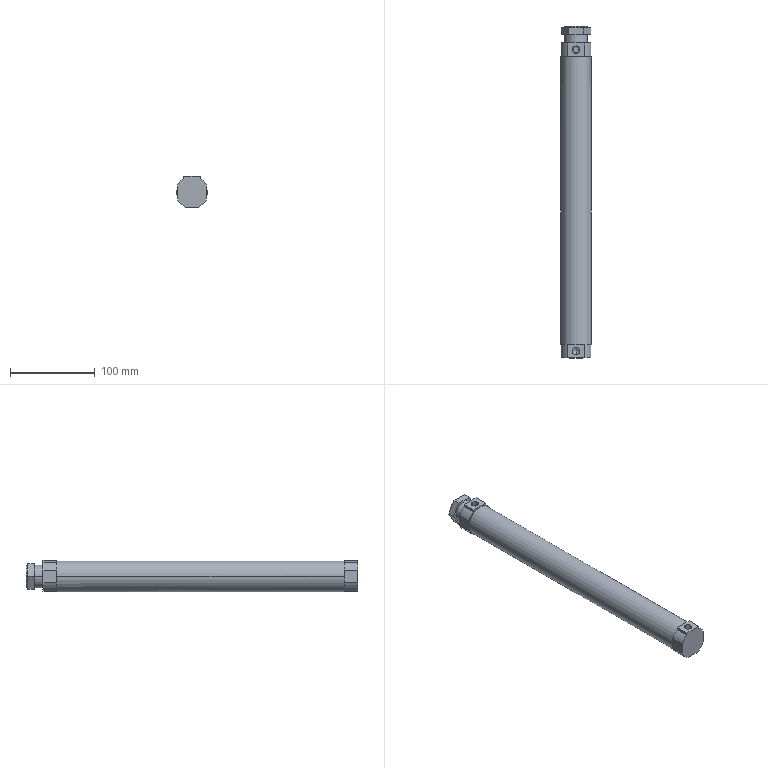Component | SolidWorks | A4-SDA 32X300-KC-L-1_A4-SDA 32X300-KC-L1-1 | 2 solids | 58 faces | box 36 x 392 x 37 mm | volume 115619 mm3 | plane 32 | cylinder 22 | cone 4 | commonest cylinder face diameters 38 x8 8.8 x4 27 x4 32 x2 36 x2 12 x2
build123d program:
from build123d import *

# Parameters (mm, degrees)
SKETCH1_R                    = 6
BOSS_EXTRUDE1_DEPTH          = 16
SKETCH2_R                    = 18
SKETCH2_R_2                  = 16
BOSS_EXTRUDE2_DEPTH          = 340
BOSS_EXTRUDE3_START          = 16
BOSS_EXTRUDE3_DEPTH          = 16
SKETCH4_R                    = 13.5
SKETCH4_R_2                  = 6
BOSS_EXTRUDE4_DEPTH          = 20
G1_8_TAPPED_HOLE1_AT_2_COUNT = 2
G1_8_TAPPED_HOLE1_AT_2_PITCH = 356
SKETCH7_R                    = 6
BOSS_EXTRUDE5_DEPTH          = 8


with BuildPart() as part:
    # Sketch1 → Boss-Extrude1 (new body)
    with BuildSketch(Plane.XY):
        with BuildLine():
            Line((-17.5, -7.399), (-17.5, 7.399))
            ThreePointArc((-17.5, 7.399), (-14.43, 12.36), (-10, 16.155))
            Line((-10, 16.155), (-10, 19))
            Line((-10, 19), (10, 19))
            Line((10, 19), (10, 16.155))
            ThreePointArc((10, 16.155), (14.43, 12.36), (17.5, 7.399))
            Line((17.5, 7.399), (17.5, -7.399))
            ThreePointArc((17.5, -7.399), (13.435, -13.435), (7.399, -17.5))
            Line((7.399, -17.5), (-7.399, -17.5))
            ThreePointArc((-7.399, -17.5), (-13.435, -13.435), (-17.5, -7.399))
        make_face()
        Circle(SKETCH1_R, mode=Mode.SUBTRACT)
    extrude(amount=BOSS_EXTRUDE1_DEPTH)

    # Sketch4 → Boss-Extrude4 (add)
    with BuildSketch(Plane.XY.offset(16)):
        Circle(SKETCH4_R)
        Circle(SKETCH4_R_2, mode=Mode.SUBTRACT)
    extrude(amount=BOSS_EXTRUDE4_DEPTH)

    # Sketch5 → G1_8 Tapped Hole1 (revolve, cut)
    with BuildSketch(Plane(origin=(0, 19, 8), x_dir=(0, 0, 1), z_dir=(1, 0, 0))):
        Polygon((0, 0), (0, 15.364), (4.4, 12.72), (4.4, 0), align=None)
    g1_8_tapped_hole1 = revolve(axis=Axis((0, 25.35, 8), (0, -1, 0)), mode=Mode.SUBTRACT)

    # Sketch7 → Boss-Extrude5 (add)
    with BuildSketch(Plane.XY.offset(26)):
        Polygon((-8.75, 15.155), (8.75, 15.155), (17.5, 0), (8.75, -15.155), (-8.75, -15.155), (-17.5, 0), align=None)
        Circle(SKETCH7_R, mode=Mode.SUBTRACT)
    extrude(amount=BOSS_EXTRUDE5_DEPTH)


with BuildPart() as body_2:
    # Sketch2 → Boss-Extrude2 (new body)
    with BuildSketch(Plane(origin=(0, 0, 0), x_dir=(-1, 0, 0), z_dir=(0, 0, -1))):
        Circle(SKETCH2_R)
        Circle(SKETCH2_R_2, mode=Mode.SUBTRACT)
    extrude(amount=BOSS_EXTRUDE2_DEPTH)

    # Sketch3 → Boss-Extrude3 (add)
    with BuildSketch(Plane(origin=(0, 0, -340), x_dir=(-1, 0, 0), z_dir=(0, 0, -1)).offset(BOSS_EXTRUDE3_START)):
        with BuildLine():
            Line((17.5, 7.399), (17.5, -7.399))
            ThreePointArc((17.5, -7.399), (13.435, -13.435), (7.399, -17.5))
            Line((7.399, -17.5), (-7.399, -17.5))
            ThreePointArc((-7.399, -17.5), (-13.435, -13.435), (-17.5, -7.399))
            Line((-17.5, -7.399), (-17.5, 7.399))
            ThreePointArc((-17.5, 7.399), (-14.43, 12.36), (-10, 16.155))
            Line((-10, 16.155), (-10, 19))
            Line((-10, 19), (10, 19))
            Line((10, 19), (10, 16.155))
            ThreePointArc((10, 16.155), (14.43, 12.36), (17.5, 7.399))
        make_face()
    extrude(amount=-BOSS_EXTRUDE3_DEPTH)

    # G1_8 Tapped Hole1 at 2: G1_8 Tapped Hole1 ×2
    with Locations(*[(0, 0, -i * G1_8_TAPPED_HOLE1_AT_2_PITCH) for i in range(1, G1_8_TAPPED_HOLE1_AT_2_COUNT)]):
        add(g1_8_tapped_hole1, mode=Mode.SUBTRACT)


solid = Compound([part.part, body_2.part])

# Placed as in the assembly
solid = solid.moved(Location((0, -16, 31), (-90, 0, 180)))